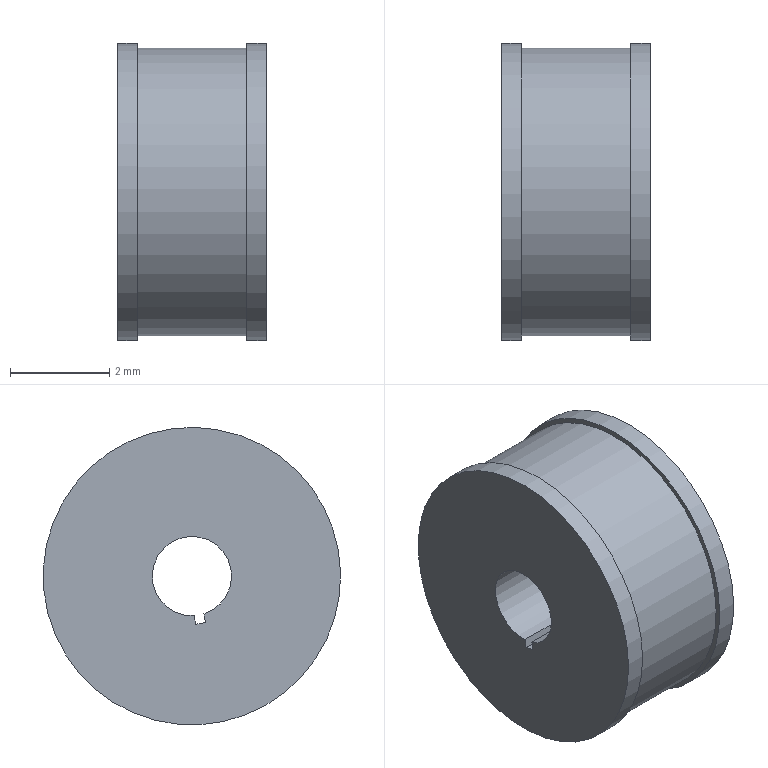Component | NX | ROUND_TRANSFER_3 | 1 solid | 11 faces | box 3 x 6 x 6 mm | volume 75 mm3 | plane 7 | cylinder 4 | commonest cylinder face diameters 6 x2 1.6 x1 5.8 x1
STEP:
#1=CARTESIAN_POINT('',(0.,0.,0.));
#2=DIRECTION('',(0.,0.,1.));
#3=DIRECTION('',(1.,0.,0.));
#4=AXIS2_PLACEMENT_3D('',#1,#2,#3);
#5=CARTESIAN_POINT('',(-47.5,-6.528,30.525));
#6=VERTEX_POINT('',#5);
#7=CARTESIAN_POINT('',(-47.5,-3.575,30.));
#8=DIRECTION('',(1.,0.,0.));
#9=DIRECTION('',(0.,-0.9846,0.175));
#10=AXIS2_PLACEMENT_3D('',#7,#8,#9);
#11=CIRCLE('',#10,3.);
#12=CARTESIAN_POINT('',(-44.5,-3.575,30.));
#13=DIRECTION('',(-1.,0.,0.));
#14=DIRECTION('',(0.,-0.175,-0.9846));
#15=AXIS2_PLACEMENT_3D('',#12,#13,#14);
#16=CYLINDRICAL_SURFACE('',#15,3.);
#17=CARTESIAN_POINT('',(7.854,3.));
#18=DIRECTION('',(-1.,0.));
#19=VECTOR('',#18,1.);
#20=LINE('',#17,#19);
#21=(GEOMETRIC_REPRESENTATION_CONTEXT(2)PARAMETRIC_REPRESENTATION_CONTEXT()REPRESENTATION_CONTEXT('',''));
#22=DEFINITIONAL_REPRESENTATION('',(#20),#21);
#23=PCURVE('',#16,#22);
#24=CARTESIAN_POINT('',(-47.5,-3.575,30.));
#25=DIRECTION('',(1.,0.,0.));
#26=DIRECTION('',(0.,0.175,0.9846));
#27=AXIS2_PLACEMENT_3D('',#24,#25,#26);
#28=PLANE('',#27);
#29=CARTESIAN_POINT('',(0.,0.));
#30=DIRECTION('',(0.,1.));
#31=AXIS2_PLACEMENT_2D('',#29,#30);
#32=CIRCLE('',#31,3.);
#33=(GEOMETRIC_REPRESENTATION_CONTEXT(2)PARAMETRIC_REPRESENTATION_CONTEXT()REPRESENTATION_CONTEXT('',''));
#34=DEFINITIONAL_REPRESENTATION('',(#32),#33);
#35=PCURVE('',#28,#34);
#36=SURFACE_CURVE('',#11,(#23,#35),.PCURVE_S1.);
#37=EDGE_CURVE('',#6,#6,#36,.T.);
#38=ORIENTED_EDGE('',*,*,#37,.T.);
#39=CARTESIAN_POINT('',(-47.1,-6.528,30.525));
#40=VERTEX_POINT('',#39);
#41=CARTESIAN_POINT('',(-47.1,-6.528,30.525));
#42=CARTESIAN_POINT('',(-47.5,-6.528,30.525));
#43=B_SPLINE_CURVE_WITH_KNOTS('',1,(#41,#42),.UNSPECIFIED.,.F.,.F.,(2,2),(2.6,3.),.PIECEWISE_BEZIER_KNOTS.);
#44=CARTESIAN_POINT('',(1.571,0.));
#45=DIRECTION('',(0.,1.));
#46=VECTOR('',#45,1.);
#47=LINE('',#44,#46);
#48=(GEOMETRIC_REPRESENTATION_CONTEXT(2)PARAMETRIC_REPRESENTATION_CONTEXT()REPRESENTATION_CONTEXT('',''));
#49=DEFINITIONAL_REPRESENTATION('',(#47),#48);
#50=PCURVE('',#16,#49);
#51=CARTESIAN_POINT('',(7.854,0.));
#52=DIRECTION('',(0.,1.));
#53=VECTOR('',#52,1.);
#54=LINE('',#51,#53);
#55=(GEOMETRIC_REPRESENTATION_CONTEXT(2)PARAMETRIC_REPRESENTATION_CONTEXT()REPRESENTATION_CONTEXT('',''));
#56=DEFINITIONAL_REPRESENTATION('',(#54),#55);
#57=PCURVE('',#16,#56);
#58=SEAM_CURVE('',#43,(#50,#57),.PCURVE_S1.);
#59=EDGE_CURVE('',#40,#6,#58,.T.);
#60=ORIENTED_EDGE('',*,*,#59,.F.);
#61=CARTESIAN_POINT('',(-47.1,-3.575,30.));
#62=DIRECTION('',(1.,0.,0.));
#63=DIRECTION('',(0.,-0.9846,0.175));
#64=AXIS2_PLACEMENT_3D('',#61,#62,#63);
#65=CIRCLE('',#64,3.);
#66=CARTESIAN_POINT('',(7.854,2.6));
#67=DIRECTION('',(-1.,0.));
#68=VECTOR('',#67,1.);
#69=LINE('',#66,#68);
#70=(GEOMETRIC_REPRESENTATION_CONTEXT(2)PARAMETRIC_REPRESENTATION_CONTEXT()REPRESENTATION_CONTEXT('',''));
#71=DEFINITIONAL_REPRESENTATION('',(#69),#70);
#72=PCURVE('',#16,#71);
#73=CARTESIAN_POINT('',(-47.1,-3.575,30.));
#74=DIRECTION('',(1.,0.,0.));
#75=DIRECTION('',(0.,0.175,0.9846));
#76=AXIS2_PLACEMENT_3D('',#73,#74,#75);
#77=PLANE('',#76);
#78=CARTESIAN_POINT('',(0.,0.));
#79=DIRECTION('',(0.,1.));
#80=AXIS2_PLACEMENT_2D('',#78,#79);
#81=CIRCLE('',#80,3.);
#82=(GEOMETRIC_REPRESENTATION_CONTEXT(2)PARAMETRIC_REPRESENTATION_CONTEXT()REPRESENTATION_CONTEXT('',''));
#83=DEFINITIONAL_REPRESENTATION('',(#81),#82);
#84=PCURVE('',#77,#83);
#85=SURFACE_CURVE('',#65,(#72,#84),.PCURVE_S1.);
#86=EDGE_CURVE('',#40,#40,#85,.T.);
#87=ORIENTED_EDGE('',*,*,#86,.F.);
#88=ORIENTED_EDGE('',*,*,#59,.T.);
#89=EDGE_LOOP('',(#38,#60,#87,#88));
#90=FACE_BOUND('',#89,.T.);
#91=ADVANCED_FACE('',(#90),#16,.T.);
#92=CARTESIAN_POINT('',(-44.9,-6.528,30.525));
#93=VERTEX_POINT('',#92);
#94=CARTESIAN_POINT('',(-44.9,-3.575,30.));
#95=DIRECTION('',(1.,0.,0.));
#96=DIRECTION('',(0.,-0.9846,0.175));
#97=AXIS2_PLACEMENT_3D('',#94,#95,#96);
#98=CIRCLE('',#97,3.);
#99=CARTESIAN_POINT('',(-44.5,-3.575,30.));
#100=DIRECTION('',(-1.,0.,0.));
#101=DIRECTION('',(0.,-0.175,-0.9846));
#102=AXIS2_PLACEMENT_3D('',#99,#100,#101);
#103=CYLINDRICAL_SURFACE('',#102,3.);
#104=CARTESIAN_POINT('',(7.854,0.4));
#105=DIRECTION('',(-1.,0.));
#106=VECTOR('',#105,1.);
#107=LINE('',#104,#106);
#108=(GEOMETRIC_REPRESENTATION_CONTEXT(2)PARAMETRIC_REPRESENTATION_CONTEXT()REPRESENTATION_CONTEXT('',''));
#109=DEFINITIONAL_REPRESENTATION('',(#107),#108);
#110=PCURVE('',#103,#109);
#111=CARTESIAN_POINT('',(-44.9,-3.575,30.));
#112=DIRECTION('',(1.,0.,0.));
#113=DIRECTION('',(0.,0.175,0.9846));
#114=AXIS2_PLACEMENT_3D('',#111,#112,#113);
#115=PLANE('',#114);
#116=CARTESIAN_POINT('',(0.,0.));
#117=DIRECTION('',(0.,1.));
#118=AXIS2_PLACEMENT_2D('',#116,#117);
#119=CIRCLE('',#118,3.);
#120=(GEOMETRIC_REPRESENTATION_CONTEXT(2)PARAMETRIC_REPRESENTATION_CONTEXT()REPRESENTATION_CONTEXT('',''));
#121=DEFINITIONAL_REPRESENTATION('',(#119),#120);
#122=PCURVE('',#115,#121);
#123=SURFACE_CURVE('',#98,(#110,#122),.PCURVE_S1.);
#124=EDGE_CURVE('',#93,#93,#123,.T.);
#125=ORIENTED_EDGE('',*,*,#124,.T.);
#126=CARTESIAN_POINT('',(-44.5,-6.528,30.525));
#127=VERTEX_POINT('',#126);
#128=CARTESIAN_POINT('',(-44.5,-6.528,30.525));
#129=CARTESIAN_POINT('',(-44.9,-6.528,30.525));
#130=B_SPLINE_CURVE_WITH_KNOTS('',1,(#128,#129),.UNSPECIFIED.,.F.,.F.,(2,2),(0.,0.4),.PIECEWISE_BEZIER_KNOTS.);
#131=CARTESIAN_POINT('',(1.571,0.));
#132=DIRECTION('',(0.,1.));
#133=VECTOR('',#132,1.);
#134=LINE('',#131,#133);
#135=(GEOMETRIC_REPRESENTATION_CONTEXT(2)PARAMETRIC_REPRESENTATION_CONTEXT()REPRESENTATION_CONTEXT('',''));
#136=DEFINITIONAL_REPRESENTATION('',(#134),#135);
#137=PCURVE('',#103,#136);
#138=CARTESIAN_POINT('',(7.854,0.));
#139=DIRECTION('',(0.,1.));
#140=VECTOR('',#139,1.);
#141=LINE('',#138,#140);
#142=(GEOMETRIC_REPRESENTATION_CONTEXT(2)PARAMETRIC_REPRESENTATION_CONTEXT()REPRESENTATION_CONTEXT('',''));
#143=DEFINITIONAL_REPRESENTATION('',(#141),#142);
#144=PCURVE('',#103,#143);
#145=SEAM_CURVE('',#130,(#137,#144),.PCURVE_S1.);
#146=EDGE_CURVE('',#127,#93,#145,.T.);
#147=ORIENTED_EDGE('',*,*,#146,.F.);
#148=CARTESIAN_POINT('',(-44.5,-3.575,30.));
#149=DIRECTION('',(1.,0.,0.));
#150=DIRECTION('',(0.,-0.9846,0.175));
#151=AXIS2_PLACEMENT_3D('',#148,#149,#150);
#152=CIRCLE('',#151,3.);
#153=CARTESIAN_POINT('',(7.854,0.));
#154=DIRECTION('',(-1.,0.));
#155=VECTOR('',#154,1.);
#156=LINE('',#153,#155);
#157=(GEOMETRIC_REPRESENTATION_CONTEXT(2)PARAMETRIC_REPRESENTATION_CONTEXT()REPRESENTATION_CONTEXT('',''));
#158=DEFINITIONAL_REPRESENTATION('',(#156),#157);
#159=PCURVE('',#103,#158);
#160=CARTESIAN_POINT('',(-44.5,-3.575,30.));
#161=DIRECTION('',(1.,0.,0.));
#162=DIRECTION('',(0.,0.175,0.9846));
#163=AXIS2_PLACEMENT_3D('',#160,#161,#162);
#164=PLANE('',#163);
#165=CARTESIAN_POINT('',(0.,0.));
#166=DIRECTION('',(0.,1.));
#167=AXIS2_PLACEMENT_2D('',#165,#166);
#168=CIRCLE('',#167,3.);
#169=(GEOMETRIC_REPRESENTATION_CONTEXT(2)PARAMETRIC_REPRESENTATION_CONTEXT()REPRESENTATION_CONTEXT('',''));
#170=DEFINITIONAL_REPRESENTATION('',(#168),#169);
#171=PCURVE('',#164,#170);
#172=SURFACE_CURVE('',#152,(#159,#171),.PCURVE_S1.);
#173=EDGE_CURVE('',#127,#127,#172,.T.);
#174=ORIENTED_EDGE('',*,*,#173,.F.);
#175=ORIENTED_EDGE('',*,*,#146,.T.);
#176=EDGE_LOOP('',(#125,#147,#174,#175));
#177=FACE_BOUND('',#176,.T.);
#178=ADVANCED_FACE('',(#177),#103,.T.);
#179=CARTESIAN_POINT('',(-47.5,-3.621,29.201));
#180=VERTEX_POINT('',#179);
#181=CARTESIAN_POINT('',(-47.5,-3.817,29.238));
#182=VERTEX_POINT('',#181);
#183=CARTESIAN_POINT('',(-47.5,-3.575,30.));
#184=DIRECTION('',(1.,0.,0.));
#185=DIRECTION('',(0.,-0.9846,0.175));
#186=AXIS2_PLACEMENT_3D('',#183,#184,#185);
#187=CIRCLE('',#186,0.8);
#188=CARTESIAN_POINT('',(-44.5,-3.575,30.));
#189=DIRECTION('',(-1.,0.,0.));
#190=DIRECTION('',(0.,-0.175,-0.9846));
#191=AXIS2_PLACEMENT_3D('',#188,#189,#190);
#192=CYLINDRICAL_SURFACE('',#191,0.8);
#193=CARTESIAN_POINT('',(7.854,3.));
#194=DIRECTION('',(-1.,0.));
#195=VECTOR('',#194,1.);
#196=LINE('',#193,#195);
#197=(GEOMETRIC_REPRESENTATION_CONTEXT(2)PARAMETRIC_REPRESENTATION_CONTEXT()REPRESENTATION_CONTEXT('',''));
#198=DEFINITIONAL_REPRESENTATION('',(#196),#197);
#199=PCURVE('',#192,#198);
#200=CARTESIAN_POINT('',(0.,0.));
#201=DIRECTION('',(-0.,1.));
#202=AXIS2_PLACEMENT_2D('',#200,#201);
#203=CIRCLE('',#202,0.8);
#204=(GEOMETRIC_REPRESENTATION_CONTEXT(2)PARAMETRIC_REPRESENTATION_CONTEXT()REPRESENTATION_CONTEXT('',''));
#205=DEFINITIONAL_REPRESENTATION('',(#203),#204);
#206=PCURVE('',#28,#205);
#207=SURFACE_CURVE('',#187,(#199,#206),.PCURVE_S1.);
#208=EDGE_CURVE('',#180,#182,#207,.T.);
#209=ORIENTED_EDGE('',*,*,#208,.T.);
#210=CARTESIAN_POINT('',(-44.5,-3.817,29.238));
#211=VERTEX_POINT('',#210);
#212=CARTESIAN_POINT('',(-44.5,-3.817,29.238));
#213=DIRECTION('',(1.,0.,0.));
#214=VECTOR('',#213,1.);
#215=LINE('',#212,#214);
#216=CARTESIAN_POINT('',(0.1324,0.));
#217=DIRECTION('',(0.,-1.));
#218=VECTOR('',#217,1.);
#219=LINE('',#216,#218);
#220=(GEOMETRIC_REPRESENTATION_CONTEXT(2)PARAMETRIC_REPRESENTATION_CONTEXT()REPRESENTATION_CONTEXT('',''));
#221=DEFINITIONAL_REPRESENTATION('',(#219),#220);
#222=PCURVE('',#192,#221);
#223=CARTESIAN_POINT('',(-93.5,-3.767,29.508));
#224=DIRECTION('',(0.,-0.9833,0.1819));
#225=DIRECTION('',(0.,-0.1819,-0.9833));
#226=AXIS2_PLACEMENT_3D('',#223,#224,#225);
#227=PLANE('',#226);
#228=CARTESIAN_POINT('',(0.275,49.));
#229=DIRECTION('',(0.,1.));
#230=VECTOR('',#229,1.);
#231=LINE('',#228,#230);
#232=(GEOMETRIC_REPRESENTATION_CONTEXT(2)PARAMETRIC_REPRESENTATION_CONTEXT()REPRESENTATION_CONTEXT('',''));
#233=DEFINITIONAL_REPRESENTATION('',(#231),#232);
#234=PCURVE('',#227,#233);
#235=SURFACE_CURVE('',#215,(#222,#234),.PCURVE_S1.);
#236=EDGE_CURVE('',#182,#211,#235,.T.);
#237=ORIENTED_EDGE('',*,*,#236,.T.);
#238=CARTESIAN_POINT('',(-44.5,-3.621,29.201));
#239=VERTEX_POINT('',#238);
#240=CARTESIAN_POINT('',(-44.5,-3.575,30.));
#241=DIRECTION('',(1.,0.,0.));
#242=DIRECTION('',(0.,-0.9846,0.175));
#243=AXIS2_PLACEMENT_3D('',#240,#241,#242);
#244=CIRCLE('',#243,0.8);
#245=CARTESIAN_POINT('',(7.854,0.));
#246=DIRECTION('',(-1.,0.));
#247=VECTOR('',#246,1.);
#248=LINE('',#245,#247);
#249=(GEOMETRIC_REPRESENTATION_CONTEXT(2)PARAMETRIC_REPRESENTATION_CONTEXT()REPRESENTATION_CONTEXT('',''));
#250=DEFINITIONAL_REPRESENTATION('',(#248),#249);
#251=PCURVE('',#192,#250);
#252=CARTESIAN_POINT('',(0.,0.));
#253=DIRECTION('',(-0.,1.));
#254=AXIS2_PLACEMENT_2D('',#252,#253);
#255=CIRCLE('',#254,0.8);
#256=(GEOMETRIC_REPRESENTATION_CONTEXT(2)PARAMETRIC_REPRESENTATION_CONTEXT()REPRESENTATION_CONTEXT('',''));
#257=DEFINITIONAL_REPRESENTATION('',(#255),#256);
#258=PCURVE('',#164,#257);
#259=SURFACE_CURVE('',#244,(#251,#258),.PCURVE_S1.);
#260=EDGE_CURVE('',#239,#211,#259,.T.);
#261=ORIENTED_EDGE('',*,*,#260,.F.);
#262=CARTESIAN_POINT('',(-44.5,-3.621,29.201));
#263=DIRECTION('',(-1.,0.,0.));
#264=VECTOR('',#263,1.);
#265=LINE('',#262,#264);
#266=CARTESIAN_POINT('',(6.165,0.));
#267=DIRECTION('',(0.,1.));
#268=VECTOR('',#267,1.);
#269=LINE('',#266,#268);
#270=(GEOMETRIC_REPRESENTATION_CONTEXT(2)PARAMETRIC_REPRESENTATION_CONTEXT()REPRESENTATION_CONTEXT('',''));
#271=DEFINITIONAL_REPRESENTATION('',(#269),#270);
#272=PCURVE('',#192,#271);
#273=CARTESIAN_POINT('',(-93.5,-3.653,29.029));
#274=DIRECTION('',(0.,0.9833,-0.1819));
#275=DIRECTION('',(0.,0.1819,0.9833));
#276=AXIS2_PLACEMENT_3D('',#273,#274,#275);
#277=PLANE('',#276);
#278=CARTESIAN_POINT('',(0.175,49.));
#279=DIRECTION('',(0.,-1.));
#280=VECTOR('',#279,1.);
#281=LINE('',#278,#280);
#282=(GEOMETRIC_REPRESENTATION_CONTEXT(2)PARAMETRIC_REPRESENTATION_CONTEXT()REPRESENTATION_CONTEXT('',''));
#283=DEFINITIONAL_REPRESENTATION('',(#281),#282);
#284=PCURVE('',#277,#283);
#285=SURFACE_CURVE('',#265,(#272,#284),.PCURVE_S1.);
#286=EDGE_CURVE('',#239,#180,#285,.T.);
#287=ORIENTED_EDGE('',*,*,#286,.T.);
#288=EDGE_LOOP('',(#209,#237,#261,#287));
#289=FACE_BOUND('',#288,.F.);
#290=ADVANCED_FACE('',(#289),#192,.F.);
#291=CARTESIAN_POINT('',(-44.5,-3.653,29.029));
#292=VERTEX_POINT('',#291);
#293=CARTESIAN_POINT('',(-44.5,-3.476,29.982));
#294=DIRECTION('',(0.,0.1819,0.9833));
#295=VECTOR('',#294,1.);
#296=LINE('',#293,#295);
#297=CARTESIAN_POINT('',(-0.0007097,-0.1));
#298=DIRECTION('',(1.,-0.007097));
#299=VECTOR('',#298,1.);
#300=LINE('',#297,#299);
#301=(GEOMETRIC_REPRESENTATION_CONTEXT(2)PARAMETRIC_REPRESENTATION_CONTEXT()REPRESENTATION_CONTEXT('',''));
#302=DEFINITIONAL_REPRESENTATION('',(#300),#301);
#303=PCURVE('',#164,#302);
#304=CARTESIAN_POINT('',(0.9687,49.));
#305=DIRECTION('',(1.,0.));
#306=VECTOR('',#305,1.);
#307=LINE('',#304,#306);
#308=(GEOMETRIC_REPRESENTATION_CONTEXT(2)PARAMETRIC_REPRESENTATION_CONTEXT()REPRESENTATION_CONTEXT('',''));
#309=DEFINITIONAL_REPRESENTATION('',(#307),#308);
#310=PCURVE('',#277,#309);
#311=SURFACE_CURVE('',#296,(#303,#310),.PCURVE_S1.);
#312=EDGE_CURVE('',#292,#239,#311,.T.);
#313=ORIENTED_EDGE('',*,*,#312,.F.);
#314=CARTESIAN_POINT('',(-44.5,-3.849,29.066));
#315=VERTEX_POINT('',#314);
#316=CARTESIAN_POINT('',(-44.5,-3.751,29.047));
#317=DIRECTION('',(0.,0.9833,-0.1819));
#318=VECTOR('',#317,1.);
#319=LINE('',#316,#318);
#320=CARTESIAN_POINT('',(-0.9687,0.006875));
#321=DIRECTION('',(-0.007097,-1.));
#322=VECTOR('',#321,1.);
#323=LINE('',#320,#322);
#324=(GEOMETRIC_REPRESENTATION_CONTEXT(2)PARAMETRIC_REPRESENTATION_CONTEXT()REPRESENTATION_CONTEXT('',''));
#325=DEFINITIONAL_REPRESENTATION('',(#323),#324);
#326=PCURVE('',#164,#325);
#327=CARTESIAN_POINT('',(-93.5,-3.849,29.066));
#328=DIRECTION('',(0.,-0.1819,-0.9833));
#329=DIRECTION('',(0.,0.9833,-0.1819));
#330=AXIS2_PLACEMENT_3D('',#327,#328,#329);
#331=PLANE('',#330);
#332=CARTESIAN_POINT('',(0.1,49.));
#333=DIRECTION('',(1.,0.));
#334=VECTOR('',#333,1.);
#335=LINE('',#332,#334);
#336=(GEOMETRIC_REPRESENTATION_CONTEXT(2)PARAMETRIC_REPRESENTATION_CONTEXT()REPRESENTATION_CONTEXT('',''));
#337=DEFINITIONAL_REPRESENTATION('',(#335),#336);
#338=PCURVE('',#331,#337);
#339=SURFACE_CURVE('',#319,(#326,#338),.PCURVE_S1.);
#340=EDGE_CURVE('',#315,#292,#339,.T.);
#341=ORIENTED_EDGE('',*,*,#340,.F.);
#342=CARTESIAN_POINT('',(-44.5,-3.673,30.018));
#343=DIRECTION('',(0.,-0.1819,-0.9833));
#344=VECTOR('',#343,1.);
#345=LINE('',#342,#344);
#346=CARTESIAN_POINT('',(0.0007097,0.1));
#347=DIRECTION('',(-1.,0.007097));
#348=VECTOR('',#347,1.);
#349=LINE('',#346,#348);
#350=(GEOMETRIC_REPRESENTATION_CONTEXT(2)PARAMETRIC_REPRESENTATION_CONTEXT()REPRESENTATION_CONTEXT('',''));
#351=DEFINITIONAL_REPRESENTATION('',(#349),#350);
#352=PCURVE('',#164,#351);
#353=CARTESIAN_POINT('',(-0.5187,49.));
#354=DIRECTION('',(1.,0.));
#355=VECTOR('',#354,1.);
#356=LINE('',#353,#355);
#357=(GEOMETRIC_REPRESENTATION_CONTEXT(2)PARAMETRIC_REPRESENTATION_CONTEXT()REPRESENTATION_CONTEXT('',''));
#358=DEFINITIONAL_REPRESENTATION('',(#356),#357);
#359=PCURVE('',#227,#358);
#360=SURFACE_CURVE('',#345,(#352,#359),.PCURVE_S1.);
#361=EDGE_CURVE('',#211,#315,#360,.T.);
#362=ORIENTED_EDGE('',*,*,#361,.F.);
#363=ORIENTED_EDGE('',*,*,#260,.F.);
#364=EDGE_LOOP('',(#313,#341,#362,#363));
#365=FACE_BOUND('',#364,.T.);
#366=ORIENTED_EDGE('',*,*,#173,.T.);
#367=EDGE_LOOP('',(#366));
#368=FACE_BOUND('',#367,.T.);
#369=ADVANCED_FACE('',(#365,#368),#164,.T.);
#370=ORIENTED_EDGE('',*,*,#37,.F.);
#371=EDGE_LOOP('',(#370));
#372=FACE_BOUND('',#371,.T.);
#373=CARTESIAN_POINT('',(-47.5,-3.849,29.066));
#374=VERTEX_POINT('',#373);
#375=CARTESIAN_POINT('',(-47.5,-3.653,29.029));
#376=VERTEX_POINT('',#375);
#377=CARTESIAN_POINT('',(-47.5,-3.751,29.047));
#378=DIRECTION('',(0.,0.9833,-0.1819));
#379=VECTOR('',#378,1.);
#380=LINE('',#377,#379);
#381=CARTESIAN_POINT('',(-0.9687,0.006875));
#382=DIRECTION('',(-0.007097,-1.));
#383=VECTOR('',#382,1.);
#384=LINE('',#381,#383);
#385=(GEOMETRIC_REPRESENTATION_CONTEXT(2)PARAMETRIC_REPRESENTATION_CONTEXT()REPRESENTATION_CONTEXT('',''));
#386=DEFINITIONAL_REPRESENTATION('',(#384),#385);
#387=PCURVE('',#28,#386);
#388=CARTESIAN_POINT('',(0.1,46.));
#389=DIRECTION('',(1.,0.));
#390=VECTOR('',#389,1.);
#391=LINE('',#388,#390);
#392=(GEOMETRIC_REPRESENTATION_CONTEXT(2)PARAMETRIC_REPRESENTATION_CONTEXT()REPRESENTATION_CONTEXT('',''));
#393=DEFINITIONAL_REPRESENTATION('',(#391),#392);
#394=PCURVE('',#331,#393);
#395=SURFACE_CURVE('',#380,(#387,#394),.PCURVE_S1.);
#396=EDGE_CURVE('',#374,#376,#395,.T.);
#397=ORIENTED_EDGE('',*,*,#396,.T.);
#398=CARTESIAN_POINT('',(-47.5,-3.476,29.982));
#399=DIRECTION('',(0.,0.1819,0.9833));
#400=VECTOR('',#399,1.);
#401=LINE('',#398,#400);
#402=CARTESIAN_POINT('',(-0.0007097,-0.1));
#403=DIRECTION('',(1.,-0.007097));
#404=VECTOR('',#403,1.);
#405=LINE('',#402,#404);
#406=(GEOMETRIC_REPRESENTATION_CONTEXT(2)PARAMETRIC_REPRESENTATION_CONTEXT()REPRESENTATION_CONTEXT('',''));
#407=DEFINITIONAL_REPRESENTATION('',(#405),#406);
#408=PCURVE('',#28,#407);
#409=CARTESIAN_POINT('',(0.9687,46.));
#410=DIRECTION('',(1.,0.));
#411=VECTOR('',#410,1.);
#412=LINE('',#409,#411);
#413=(GEOMETRIC_REPRESENTATION_CONTEXT(2)PARAMETRIC_REPRESENTATION_CONTEXT()REPRESENTATION_CONTEXT('',''));
#414=DEFINITIONAL_REPRESENTATION('',(#412),#413);
#415=PCURVE('',#277,#414);
#416=SURFACE_CURVE('',#401,(#408,#415),.PCURVE_S1.);
#417=EDGE_CURVE('',#376,#180,#416,.T.);
#418=ORIENTED_EDGE('',*,*,#417,.T.);
#419=ORIENTED_EDGE('',*,*,#208,.T.);
#420=CARTESIAN_POINT('',(-47.5,-3.673,30.018));
#421=DIRECTION('',(0.,-0.1819,-0.9833));
#422=VECTOR('',#421,1.);
#423=LINE('',#420,#422);
#424=CARTESIAN_POINT('',(0.0007097,0.1));
#425=DIRECTION('',(-1.,0.007097));
#426=VECTOR('',#425,1.);
#427=LINE('',#424,#426);
#428=(GEOMETRIC_REPRESENTATION_CONTEXT(2)PARAMETRIC_REPRESENTATION_CONTEXT()REPRESENTATION_CONTEXT('',''));
#429=DEFINITIONAL_REPRESENTATION('',(#427),#428);
#430=PCURVE('',#28,#429);
#431=CARTESIAN_POINT('',(-0.5187,46.));
#432=DIRECTION('',(1.,0.));
#433=VECTOR('',#432,1.);
#434=LINE('',#431,#433);
#435=(GEOMETRIC_REPRESENTATION_CONTEXT(2)PARAMETRIC_REPRESENTATION_CONTEXT()REPRESENTATION_CONTEXT('',''));
#436=DEFINITIONAL_REPRESENTATION('',(#434),#435);
#437=PCURVE('',#227,#436);
#438=SURFACE_CURVE('',#423,(#430,#437),.PCURVE_S1.);
#439=EDGE_CURVE('',#182,#374,#438,.T.);
#440=ORIENTED_EDGE('',*,*,#439,.T.);
#441=EDGE_LOOP('',(#397,#418,#419,#440));
#442=FACE_BOUND('',#441,.T.);
#443=ADVANCED_FACE('',(#372,#442),#28,.F.);
#444=CARTESIAN_POINT('',(-44.9,-6.43,30.507));
#445=VERTEX_POINT('',#444);
#446=CARTESIAN_POINT('',(-44.9,-3.575,30.));
#447=DIRECTION('',(-1.,0.,0.));
#448=DIRECTION('',(0.,-0.9846,0.175));
#449=AXIS2_PLACEMENT_3D('',#446,#447,#448);
#450=CIRCLE('',#449,2.9);
#451=CARTESIAN_POINT('',(-44.9,-3.575,30.));
#452=DIRECTION('',(-1.,0.,0.));
#453=DIRECTION('',(0.,-0.175,-0.9846));
#454=AXIS2_PLACEMENT_3D('',#451,#452,#453);
#455=CYLINDRICAL_SURFACE('',#454,2.9);
#456=CARTESIAN_POINT('',(1.571,0.));
#457=DIRECTION('',(1.,0.));
#458=VECTOR('',#457,1.);
#459=LINE('',#456,#458);
#460=(GEOMETRIC_REPRESENTATION_CONTEXT(2)PARAMETRIC_REPRESENTATION_CONTEXT()REPRESENTATION_CONTEXT('',''));
#461=DEFINITIONAL_REPRESENTATION('',(#459),#460);
#462=PCURVE('',#455,#461);
#463=CARTESIAN_POINT('',(-0.,2.9));
#464=CARTESIAN_POINT('',(5.023,2.9));
#465=CARTESIAN_POINT('',(2.511,-1.45));
#466=CARTESIAN_POINT('',(0.,-5.8));
#467=CARTESIAN_POINT('',(-2.511,-1.45));
#468=CARTESIAN_POINT('',(-5.023,2.9));
#469=CARTESIAN_POINT('',(-0.,2.9));
#470=(BOUNDED_CURVE()B_SPLINE_CURVE(2,(#463,#464,#465,#466,#467,#468,#469),.UNSPECIFIED.,.T.,.F.)B_SPLINE_CURVE_WITH_KNOTS((1,2,2,2,2,1),(-2.094,0.,2.094,4.189,6.283,8.378),.UNSPECIFIED.)CURVE()GEOMETRIC_REPRESENTATION_ITEM()RATIONAL_B_SPLINE_CURVE((1.,0.5,1.,0.5,1.,0.5,1.))REPRESENTATION_ITEM(''));
#471=(GEOMETRIC_REPRESENTATION_CONTEXT(2)PARAMETRIC_REPRESENTATION_CONTEXT()REPRESENTATION_CONTEXT('',''));
#472=DEFINITIONAL_REPRESENTATION('',(#470),#471);
#473=PCURVE('',#115,#472);
#474=SURFACE_CURVE('',#450,(#462,#473),.PCURVE_S1.);
#475=EDGE_CURVE('',#445,#445,#474,.T.);
#476=ORIENTED_EDGE('',*,*,#475,.T.);
#477=CARTESIAN_POINT('',(-47.1,-6.43,30.507));
#478=VERTEX_POINT('',#477);
#479=CARTESIAN_POINT('',(-44.9,-6.43,30.507));
#480=CARTESIAN_POINT('',(-47.1,-6.43,30.507));
#481=B_SPLINE_CURVE_WITH_KNOTS('',1,(#479,#480),.UNSPECIFIED.,.F.,.F.,(2,2),(0.,2.2),.PIECEWISE_BEZIER_KNOTS.);
#482=CARTESIAN_POINT('',(7.854,0.));
#483=DIRECTION('',(0.,1.));
#484=VECTOR('',#483,1.);
#485=LINE('',#482,#484);
#486=(GEOMETRIC_REPRESENTATION_CONTEXT(2)PARAMETRIC_REPRESENTATION_CONTEXT()REPRESENTATION_CONTEXT('',''));
#487=DEFINITIONAL_REPRESENTATION('',(#485),#486);
#488=PCURVE('',#455,#487);
#489=CARTESIAN_POINT('',(1.571,0.));
#490=DIRECTION('',(0.,1.));
#491=VECTOR('',#490,1.);
#492=LINE('',#489,#491);
#493=(GEOMETRIC_REPRESENTATION_CONTEXT(2)PARAMETRIC_REPRESENTATION_CONTEXT()REPRESENTATION_CONTEXT('',''));
#494=DEFINITIONAL_REPRESENTATION('',(#492),#493);
#495=PCURVE('',#455,#494);
#496=SEAM_CURVE('',#481,(#488,#495),.PCURVE_S1.);
#497=EDGE_CURVE('',#445,#478,#496,.T.);
#498=ORIENTED_EDGE('',*,*,#497,.T.);
#499=CARTESIAN_POINT('',(-47.1,-3.575,30.));
#500=DIRECTION('',(-1.,0.,0.));
#501=DIRECTION('',(0.,-0.9846,0.175));
#502=AXIS2_PLACEMENT_3D('',#499,#500,#501);
#503=CIRCLE('',#502,2.9);
#504=CARTESIAN_POINT('',(1.571,2.2));
#505=DIRECTION('',(1.,0.));
#506=VECTOR('',#505,1.);
#507=LINE('',#504,#506);
#508=(GEOMETRIC_REPRESENTATION_CONTEXT(2)PARAMETRIC_REPRESENTATION_CONTEXT()REPRESENTATION_CONTEXT('',''));
#509=DEFINITIONAL_REPRESENTATION('',(#507),#508);
#510=PCURVE('',#455,#509);
#511=CARTESIAN_POINT('',(-0.,2.9));
#512=CARTESIAN_POINT('',(5.023,2.9));
#513=CARTESIAN_POINT('',(2.511,-1.45));
#514=CARTESIAN_POINT('',(0.,-5.8));
#515=CARTESIAN_POINT('',(-2.511,-1.45));
#516=CARTESIAN_POINT('',(-5.023,2.9));
#517=CARTESIAN_POINT('',(-0.,2.9));
#518=(BOUNDED_CURVE()B_SPLINE_CURVE(2,(#511,#512,#513,#514,#515,#516,#517),.UNSPECIFIED.,.T.,.F.)B_SPLINE_CURVE_WITH_KNOTS((1,2,2,2,2,1),(-2.094,0.,2.094,4.189,6.283,8.378),.UNSPECIFIED.)CURVE()GEOMETRIC_REPRESENTATION_ITEM()RATIONAL_B_SPLINE_CURVE((1.,0.5,1.,0.5,1.,0.5,1.))REPRESENTATION_ITEM(''));
#519=(GEOMETRIC_REPRESENTATION_CONTEXT(2)PARAMETRIC_REPRESENTATION_CONTEXT()REPRESENTATION_CONTEXT('',''));
#520=DEFINITIONAL_REPRESENTATION('',(#518),#519);
#521=PCURVE('',#77,#520);
#522=SURFACE_CURVE('',#503,(#510,#521),.PCURVE_S1.);
#523=EDGE_CURVE('',#478,#478,#522,.T.);
#524=ORIENTED_EDGE('',*,*,#523,.F.);
#525=ORIENTED_EDGE('',*,*,#497,.F.);
#526=EDGE_LOOP('',(#476,#498,#524,#525));
#527=FACE_BOUND('',#526,.T.);
#528=ADVANCED_FACE('',(#527),#455,.T.);
#529=ORIENTED_EDGE('',*,*,#124,.F.);
#530=EDGE_LOOP('',(#529));
#531=FACE_BOUND('',#530,.T.);
#532=ORIENTED_EDGE('',*,*,#475,.F.);
#533=EDGE_LOOP('',(#532));
#534=FACE_BOUND('',#533,.T.);
#535=ADVANCED_FACE('',(#531,#534),#115,.F.);
#536=ORIENTED_EDGE('',*,*,#86,.T.);
#537=EDGE_LOOP('',(#536));
#538=FACE_BOUND('',#537,.T.);
#539=ORIENTED_EDGE('',*,*,#523,.T.);
#540=EDGE_LOOP('',(#539));
#541=FACE_BOUND('',#540,.T.);
#542=ADVANCED_FACE('',(#538,#541),#77,.T.);
#543=ORIENTED_EDGE('',*,*,#340,.T.);
#544=CARTESIAN_POINT('',(-93.5,-3.653,29.029));
#545=DIRECTION('',(-1.,0.,0.));
#546=VECTOR('',#545,1.);
#547=LINE('',#544,#546);
#548=CARTESIAN_POINT('',(0.2,0.));
#549=DIRECTION('',(0.,-1.));
#550=VECTOR('',#549,1.);
#551=LINE('',#548,#550);
#552=(GEOMETRIC_REPRESENTATION_CONTEXT(2)PARAMETRIC_REPRESENTATION_CONTEXT()REPRESENTATION_CONTEXT('',''));
#553=DEFINITIONAL_REPRESENTATION('',(#551),#552);
#554=PCURVE('',#331,#553);
#555=CARTESIAN_POINT('',(0.,0.));
#556=DIRECTION('',(0.,-1.));
#557=VECTOR('',#556,1.);
#558=LINE('',#555,#557);
#559=(GEOMETRIC_REPRESENTATION_CONTEXT(2)PARAMETRIC_REPRESENTATION_CONTEXT()REPRESENTATION_CONTEXT('',''));
#560=DEFINITIONAL_REPRESENTATION('',(#558),#559);
#561=PCURVE('',#277,#560);
#562=SURFACE_CURVE('',#547,(#554,#561),.PCURVE_S1.);
#563=EDGE_CURVE('',#292,#376,#562,.T.);
#564=ORIENTED_EDGE('',*,*,#563,.T.);
#565=ORIENTED_EDGE('',*,*,#396,.F.);
#566=CARTESIAN_POINT('',(-93.5,-3.849,29.066));
#567=DIRECTION('',(-1.,0.,0.));
#568=VECTOR('',#567,1.);
#569=LINE('',#566,#568);
#570=CARTESIAN_POINT('',(0.,0.));
#571=DIRECTION('',(0.,-1.));
#572=VECTOR('',#571,1.);
#573=LINE('',#570,#572);
#574=(GEOMETRIC_REPRESENTATION_CONTEXT(2)PARAMETRIC_REPRESENTATION_CONTEXT()REPRESENTATION_CONTEXT('',''));
#575=DEFINITIONAL_REPRESENTATION('',(#573),#574);
#576=PCURVE('',#331,#575);
#577=CARTESIAN_POINT('',(0.45,0.));
#578=DIRECTION('',(0.,-1.));
#579=VECTOR('',#578,1.);
#580=LINE('',#577,#579);
#581=(GEOMETRIC_REPRESENTATION_CONTEXT(2)PARAMETRIC_REPRESENTATION_CONTEXT()REPRESENTATION_CONTEXT('',''));
#582=DEFINITIONAL_REPRESENTATION('',(#580),#581);
#583=PCURVE('',#227,#582);
#584=SURFACE_CURVE('',#569,(#576,#583),.PCURVE_S1.);
#585=EDGE_CURVE('',#315,#374,#584,.T.);
#586=ORIENTED_EDGE('',*,*,#585,.F.);
#587=EDGE_LOOP('',(#543,#564,#565,#586));
#588=FACE_BOUND('',#587,.T.);
#589=ADVANCED_FACE('',(#588),#331,.F.);
#590=ORIENTED_EDGE('',*,*,#312,.T.);
#591=ORIENTED_EDGE('',*,*,#286,.T.);
#592=ORIENTED_EDGE('',*,*,#417,.F.);
#593=ORIENTED_EDGE('',*,*,#563,.F.);
#594=EDGE_LOOP('',(#590,#591,#592,#593));
#595=FACE_BOUND('',#594,.T.);
#596=ADVANCED_FACE('',(#595),#277,.F.);
#597=ORIENTED_EDGE('',*,*,#361,.T.);
#598=ORIENTED_EDGE('',*,*,#585,.T.);
#599=ORIENTED_EDGE('',*,*,#439,.F.);
#600=ORIENTED_EDGE('',*,*,#236,.T.);
#601=EDGE_LOOP('',(#597,#598,#599,#600));
#602=FACE_BOUND('',#601,.T.);
#603=ADVANCED_FACE('',(#602),#227,.F.);
#604=CLOSED_SHELL('',(#91,#178,#290,#369,#443,#528,#535,#542,#589,#596,#603));
#605=MANIFOLD_SOLID_BREP('',#604);
#606=(LENGTH_UNIT()NAMED_UNIT(*)SI_UNIT(.MILLI.,.METRE.));
#607=UNCERTAINTY_MEASURE_WITH_UNIT(LENGTH_MEASURE(0.000002),#606,'','');
#608=(NAMED_UNIT(*)PLANE_ANGLE_UNIT()SI_UNIT($,.RADIAN.));
#609=(NAMED_UNIT(*)SI_UNIT($,.STERADIAN.)SOLID_ANGLE_UNIT());
#610=(GEOMETRIC_REPRESENTATION_CONTEXT(3)GLOBAL_UNCERTAINTY_ASSIGNED_CONTEXT((#607))GLOBAL_UNIT_ASSIGNED_CONTEXT((#606,#608,#609))REPRESENTATION_CONTEXT('',''));
#611=ADVANCED_BREP_SHAPE_REPRESENTATION('',(#4,#605),#610);